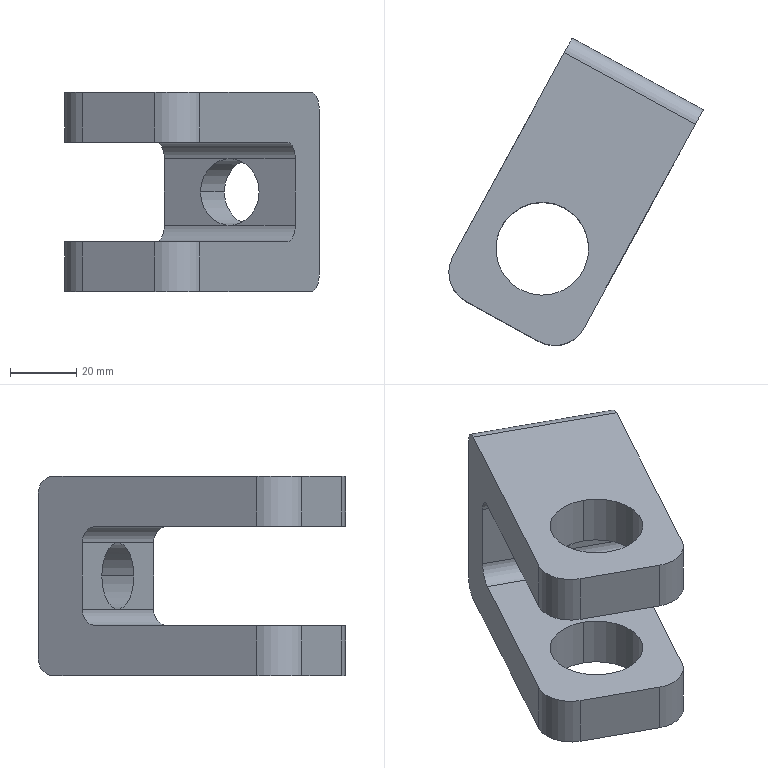Component | SolidWorks | SC-80X130-S-BCylinderY-Joint-1 | 1 solid | 25 faces | box 76.65 x 92.6 x 60 mm | volume 110480 mm3 | cylinder 14 | plane 11 | commonest cylinder face diameters 28 x4 10 x4 20 x4 20.1 x2
STEP:
#1=CARTESIAN_POINT('',(-14.174,0.0304,35.433));
#2=VERTEX_POINT('',#1);
#3=CARTESIAN_POINT('',(-13.862,-0.1403,35.827));
#4=VERTEX_POINT('',#3);
#5=CARTESIAN_POINT('',(-13.827,-0.1591,35.433));
#6=DIRECTION('',(0.479,0.8778,0.));
#7=DIRECTION('',(0.8778,-0.479,0.));
#8=AXIS2_PLACEMENT_3D('',#5,#6,#7);
#9=CIRCLE('',#8,0.3957);
#10=EDGE_CURVE('',#2,#4,#9,.T.);
#11=ORIENTED_EDGE('',*,*,#10,.F.);
#12=CARTESIAN_POINT('',(-13.892,0.5488,35.433));
#13=VERTEX_POINT('',#12);
#14=CARTESIAN_POINT('',(-13.892,0.5488,35.433));
#15=DIRECTION('',(0.479,0.8778,0.));
#16=VECTOR('',#15,39.37);
#17=LINE('',#14,#16);
#18=EDGE_CURVE('',#2,#13,#17,.T.);
#19=ORIENTED_EDGE('',*,*,#18,.T.);
#20=CARTESIAN_POINT('',(-13.197,0.1697,35.433));
#21=VERTEX_POINT('',#20);
#22=CARTESIAN_POINT('',(-13.544,0.3593,35.433));
#23=DIRECTION('',(0.479,0.8778,0.));
#24=DIRECTION('',(0.8778,-0.479,0.));
#25=AXIS2_PLACEMENT_3D('',#22,#23,#24);
#26=CIRCLE('',#25,0.3957);
#27=EDGE_CURVE('',#13,#21,#26,.T.);
#28=ORIENTED_EDGE('',*,*,#27,.T.);
#29=CARTESIAN_POINT('',(-13.48,-0.3487,35.433));
#30=VERTEX_POINT('',#29);
#31=CARTESIAN_POINT('',(-13.197,0.1697,35.433));
#32=DIRECTION('',(0.479,0.8778,0.));
#33=VECTOR('',#32,39.37);
#34=LINE('',#31,#33);
#35=EDGE_CURVE('',#30,#21,#34,.T.);
#36=ORIENTED_EDGE('',*,*,#35,.F.);
#37=CARTESIAN_POINT('',(-13.793,-0.178,35.827));
#38=VERTEX_POINT('',#37);
#39=CARTESIAN_POINT('',(-13.827,-0.1591,35.433));
#40=DIRECTION('',(0.479,0.8778,0.));
#41=DIRECTION('',(0.8778,-0.479,0.));
#42=AXIS2_PLACEMENT_3D('',#39,#40,#41);
#43=CIRCLE('',#42,0.3957);
#44=EDGE_CURVE('',#38,#30,#43,.T.);
#45=ORIENTED_EDGE('',*,*,#44,.F.);
#46=CARTESIAN_POINT('',(-13.862,-0.1403,35.827));
#47=CARTESIAN_POINT('',(-13.839,-0.1528,35.829));
#48=CARTESIAN_POINT('',(-13.816,-0.1654,35.829));
#49=CARTESIAN_POINT('',(-13.793,-0.178,35.827));
#50=B_SPLINE_CURVE_WITH_KNOTS('',3,(#46,#47,#48,#49),.UNSPECIFIED.,.F.,.F.,(4,4),(0.,0.002002),.UNSPECIFIED.);
#51=EDGE_CURVE('',#4,#38,#50,.T.);
#52=ORIENTED_EDGE('',*,*,#51,.F.);
#53=EDGE_LOOP('',(#11,#19,#28,#36,#45,#52));
#54=FACE_OUTER_BOUND('',#53,.T.);
#55=CARTESIAN_POINT('',(-13.544,0.3593,35.433));
#56=DIRECTION('',(0.479,0.8778,0.));
#57=DIRECTION('',(0.8778,-0.479,0.));
#58=AXIS2_PLACEMENT_3D('',#55,#56,#57);
#59=CYLINDRICAL_SURFACE('',#58,0.3957);
#60=ADVANCED_FACE('',(#54),#59,.F.);
#61=CARTESIAN_POINT('',(-14.94,-2.198,34.843));
#62=VERTEX_POINT('',#61);
#63=CARTESIAN_POINT('',(-14.412,-1.23,34.843));
#64=VERTEX_POINT('',#63);
#65=CARTESIAN_POINT('',(-14.676,-1.714,34.843));
#66=DIRECTION('',(-0.,0.,-1.));
#67=DIRECTION('',(0.479,0.8778,0.));
#68=AXIS2_PLACEMENT_3D('',#65,#66,#67);
#69=CIRCLE('',#68,0.5512);
#70=EDGE_CURVE('',#62,#64,#69,.T.);
#71=ORIENTED_EDGE('',*,*,#70,.F.);
#72=CARTESIAN_POINT('',(-14.94,-2.198,34.252));
#73=VERTEX_POINT('',#72);
#74=CARTESIAN_POINT('',(-14.94,-2.198,36.614));
#75=DIRECTION('',(-0.,0.,-1.));
#76=VECTOR('',#75,39.37);
#77=LINE('',#74,#76);
#78=EDGE_CURVE('',#62,#73,#77,.T.);
#79=ORIENTED_EDGE('',*,*,#78,.T.);
#80=CARTESIAN_POINT('',(-14.412,-1.23,34.252));
#81=VERTEX_POINT('',#80);
#82=CARTESIAN_POINT('',(-14.676,-1.714,34.252));
#83=DIRECTION('',(-0.,0.,-1.));
#84=DIRECTION('',(0.479,0.8778,0.));
#85=AXIS2_PLACEMENT_3D('',#82,#83,#84);
#86=CIRCLE('',#85,0.5512);
#87=EDGE_CURVE('',#73,#81,#86,.T.);
#88=ORIENTED_EDGE('',*,*,#87,.T.);
#89=CARTESIAN_POINT('',(-14.412,-1.23,36.614));
#90=DIRECTION('',(-0.,0.,-1.));
#91=VECTOR('',#90,39.37);
#92=LINE('',#89,#91);
#93=EDGE_CURVE('',#64,#81,#92,.T.);
#94=ORIENTED_EDGE('',*,*,#93,.F.);
#95=EDGE_LOOP('',(#71,#79,#88,#94));
#96=FACE_OUTER_BOUND('',#95,.T.);
#97=CARTESIAN_POINT('',(-14.676,-1.714,36.614));
#98=DIRECTION('',(-0.,0.,-1.));
#99=DIRECTION('',(0.479,0.8778,0.));
#100=AXIS2_PLACEMENT_3D('',#97,#98,#99);
#101=CYLINDRICAL_SURFACE('',#100,0.5512);
#102=ADVANCED_FACE('',(#96),#101,.F.);
#103=CARTESIAN_POINT('',(-14.94,-2.198,36.614));
#104=VERTEX_POINT('',#103);
#105=CARTESIAN_POINT('',(-14.412,-1.23,36.614));
#106=VERTEX_POINT('',#105);
#107=CARTESIAN_POINT('',(-14.676,-1.714,36.614));
#108=DIRECTION('',(-0.,0.,-1.));
#109=DIRECTION('',(0.479,0.8778,0.));
#110=AXIS2_PLACEMENT_3D('',#107,#108,#109);
#111=CIRCLE('',#110,0.5512);
#112=EDGE_CURVE('',#104,#106,#111,.T.);
#113=ORIENTED_EDGE('',*,*,#112,.F.);
#114=CARTESIAN_POINT('',(-14.94,-2.198,36.024));
#115=VERTEX_POINT('',#114);
#116=CARTESIAN_POINT('',(-14.94,-2.198,36.614));
#117=DIRECTION('',(-0.,0.,-1.));
#118=VECTOR('',#117,39.37);
#119=LINE('',#116,#118);
#120=EDGE_CURVE('',#104,#115,#119,.T.);
#121=ORIENTED_EDGE('',*,*,#120,.T.);
#122=CARTESIAN_POINT('',(-14.412,-1.23,36.024));
#123=VERTEX_POINT('',#122);
#124=CARTESIAN_POINT('',(-14.676,-1.714,36.024));
#125=DIRECTION('',(0.,-0.,1.));
#126=DIRECTION('',(-0.479,-0.8778,0.));
#127=AXIS2_PLACEMENT_3D('',#124,#125,#126);
#128=CIRCLE('',#127,0.5512);
#129=EDGE_CURVE('',#123,#115,#128,.T.);
#130=ORIENTED_EDGE('',*,*,#129,.F.);
#131=CARTESIAN_POINT('',(-14.412,-1.23,36.614));
#132=DIRECTION('',(-0.,0.,-1.));
#133=VECTOR('',#132,39.37);
#134=LINE('',#131,#133);
#135=EDGE_CURVE('',#106,#123,#134,.T.);
#136=ORIENTED_EDGE('',*,*,#135,.F.);
#137=EDGE_LOOP('',(#113,#121,#130,#136));
#138=FACE_OUTER_BOUND('',#137,.T.);
#139=CARTESIAN_POINT('',(-14.676,-1.714,36.614));
#140=DIRECTION('',(-0.,0.,-1.));
#141=DIRECTION('',(0.479,0.8778,0.));
#142=AXIS2_PLACEMENT_3D('',#139,#140,#141);
#143=CYLINDRICAL_SURFACE('',#142,0.5512);
#144=ADVANCED_FACE('',(#138),#143,.F.);
#145=CARTESIAN_POINT('',(-14.605,0.2652,35.039));
#146=VERTEX_POINT('',#145);
#147=CARTESIAN_POINT('',(-13.862,-0.1403,35.039));
#148=VERTEX_POINT('',#147);
#149=CARTESIAN_POINT('',(-13.05,-0.5835,35.039));
#150=DIRECTION('',(0.8778,-0.479,-0.));
#151=VECTOR('',#150,39.37);
#152=LINE('',#149,#151);
#153=EDGE_CURVE('',#146,#148,#152,.T.);
#154=ORIENTED_EDGE('',*,*,#153,.T.);
#155=CARTESIAN_POINT('',(-13.827,-0.1591,35.433));
#156=DIRECTION('',(0.479,0.8778,0.));
#157=DIRECTION('',(0.8778,-0.479,0.));
#158=AXIS2_PLACEMENT_3D('',#155,#156,#157);
#159=CIRCLE('',#158,0.3957);
#160=EDGE_CURVE('',#148,#2,#159,.T.);
#161=ORIENTED_EDGE('',*,*,#160,.T.);
#162=ORIENTED_EDGE('',*,*,#10,.T.);
#163=CARTESIAN_POINT('',(-14.605,0.2652,35.827));
#164=VERTEX_POINT('',#163);
#165=CARTESIAN_POINT('',(-14.605,0.2652,35.827));
#166=DIRECTION('',(-0.8778,0.479,0.));
#167=VECTOR('',#166,39.37);
#168=LINE('',#165,#167);
#169=EDGE_CURVE('',#4,#164,#168,.T.);
#170=ORIENTED_EDGE('',*,*,#169,.T.);
#171=CARTESIAN_POINT('',(-14.605,0.2652,34.843));
#172=DIRECTION('',(-0.,0.,-1.));
#173=VECTOR('',#172,39.37);
#174=LINE('',#171,#173);
#175=EDGE_CURVE('',#164,#146,#174,.T.);
#176=ORIENTED_EDGE('',*,*,#175,.T.);
#177=EDGE_LOOP('',(#154,#161,#162,#170,#176));
#178=FACE_OUTER_BOUND('',#177,.T.);
#179=CARTESIAN_POINT('',(-13.05,-0.5835,34.843));
#180=DIRECTION('',(0.479,0.8778,0.));
#181=DIRECTION('',(0.8778,-0.479,-0.));
#182=AXIS2_PLACEMENT_3D('',#179,#180,#181);
#183=PLANE('',#182);
#184=ADVANCED_FACE('',(#178),#183,.F.);
#185=CARTESIAN_POINT('',(-14.715,-2.814,36.024));
#186=VERTEX_POINT('',#185);
#187=CARTESIAN_POINT('',(-15.579,-2.343,36.024));
#188=VERTEX_POINT('',#187);
#189=CARTESIAN_POINT('',(-14.37,-3.003,36.024));
#190=DIRECTION('',(-0.8778,0.479,0.));
#191=VECTOR('',#190,39.37);
#192=LINE('',#189,#191);
#193=EDGE_CURVE('',#186,#188,#192,.T.);
#194=ORIENTED_EDGE('',*,*,#193,.F.);
#195=CARTESIAN_POINT('',(-14.715,-2.814,36.614));
#196=VERTEX_POINT('',#195);
#197=CARTESIAN_POINT('',(-14.715,-2.814,36.024));
#198=DIRECTION('',(0.,-0.,1.));
#199=VECTOR('',#198,39.37);
#200=LINE('',#197,#199);
#201=EDGE_CURVE('',#186,#196,#200,.T.);
#202=ORIENTED_EDGE('',*,*,#201,.T.);
#203=CARTESIAN_POINT('',(-15.579,-2.343,36.614));
#204=VERTEX_POINT('',#203);
#205=CARTESIAN_POINT('',(-14.37,-3.003,36.614));
#206=DIRECTION('',(-0.8778,0.479,0.));
#207=VECTOR('',#206,39.37);
#208=LINE('',#205,#207);
#209=EDGE_CURVE('',#196,#204,#208,.T.);
#210=ORIENTED_EDGE('',*,*,#209,.T.);
#211=CARTESIAN_POINT('',(-15.579,-2.343,36.024));
#212=DIRECTION('',(-0.,0.,-1.));
#213=VECTOR('',#212,39.37);
#214=LINE('',#211,#213);
#215=EDGE_CURVE('',#204,#188,#214,.T.);
#216=ORIENTED_EDGE('',*,*,#215,.T.);
#217=EDGE_LOOP('',(#194,#202,#210,#216));
#218=FACE_OUTER_BOUND('',#217,.T.);
#219=CARTESIAN_POINT('',(-14.37,-3.003,36.024));
#220=DIRECTION('',(0.479,0.8778,0.));
#221=DIRECTION('',(0.,-0.,1.));
#222=AXIS2_PLACEMENT_3D('',#219,#220,#221);
#223=PLANE('',#222);
#224=ADVANCED_FACE('',(#218),#223,.F.);
#225=ORIENTED_EDGE('',*,*,#129,.T.);
#226=CARTESIAN_POINT('',(-14.676,-1.714,36.024));
#227=DIRECTION('',(0.,-0.,1.));
#228=DIRECTION('',(-0.479,-0.8778,0.));
#229=AXIS2_PLACEMENT_3D('',#226,#227,#228);
#230=CIRCLE('',#229,0.5512);
#231=EDGE_CURVE('',#115,#123,#230,.T.);
#232=ORIENTED_EDGE('',*,*,#231,.T.);
#233=EDGE_LOOP('',(#225,#232));
#234=FACE_BOUND('',#233,.T.);
#235=CARTESIAN_POINT('',(-14.181,-2.657,36.024));
#236=VERTEX_POINT('',#235);
#237=CARTESIAN_POINT('',(-13.144,-0.7563,36.024));
#238=VERTEX_POINT('',#237);
#239=CARTESIAN_POINT('',(-13.05,-0.5835,36.024));
#240=DIRECTION('',(0.479,0.8778,0.));
#241=VECTOR('',#240,39.37);
#242=LINE('',#239,#241);
#243=EDGE_CURVE('',#236,#238,#242,.T.);
#244=ORIENTED_EDGE('',*,*,#243,.F.);
#245=CARTESIAN_POINT('',(-14.527,-2.468,36.024));
#246=DIRECTION('',(-0.,0.,-1.));
#247=DIRECTION('',(-0.479,-0.8778,0.));
#248=AXIS2_PLACEMENT_3D('',#245,#246,#247);
#249=CIRCLE('',#248,0.3937);
#250=EDGE_CURVE('',#236,#186,#249,.T.);
#251=ORIENTED_EDGE('',*,*,#250,.T.);
#252=ORIENTED_EDGE('',*,*,#193,.T.);
#253=CARTESIAN_POINT('',(-15.736,-1.808,36.024));
#254=VERTEX_POINT('',#253);
#255=CARTESIAN_POINT('',(-15.391,-1.997,36.024));
#256=DIRECTION('',(-0.,0.,-1.));
#257=DIRECTION('',(-0.479,-0.8778,0.));
#258=AXIS2_PLACEMENT_3D('',#255,#256,#257);
#259=CIRCLE('',#258,0.3937);
#260=EDGE_CURVE('',#188,#254,#259,.T.);
#261=ORIENTED_EDGE('',*,*,#260,.T.);
#262=CARTESIAN_POINT('',(-14.699,0.09241,36.024));
#263=VERTEX_POINT('',#262);
#264=CARTESIAN_POINT('',(-14.605,0.2652,36.024));
#265=DIRECTION('',(0.479,0.8778,0.));
#266=VECTOR('',#265,39.37);
#267=LINE('',#264,#266);
#268=EDGE_CURVE('',#254,#263,#267,.T.);
#269=ORIENTED_EDGE('',*,*,#268,.T.);
#270=CARTESIAN_POINT('',(-13.144,-0.7563,36.024));
#271=DIRECTION('',(0.8778,-0.479,-0.));
#272=VECTOR('',#271,39.37);
#273=LINE('',#270,#272);
#274=EDGE_CURVE('',#263,#238,#273,.T.);
#275=ORIENTED_EDGE('',*,*,#274,.T.);
#276=EDGE_LOOP('',(#244,#251,#252,#261,#269,#275));
#277=FACE_OUTER_BOUND('',#276,.T.);
#278=CARTESIAN_POINT('',(-13.05,-0.5835,36.024));
#279=DIRECTION('',(0.,-0.,1.));
#280=DIRECTION('',(-0.479,-0.8778,-0.));
#281=AXIS2_PLACEMENT_3D('',#278,#279,#280);
#282=PLANE('',#281);
#283=ADVANCED_FACE('',(#234,#277),#282,.F.);
#284=CARTESIAN_POINT('',(-13.05,-0.5835,35.827));
#285=VERTEX_POINT('',#284);
#286=CARTESIAN_POINT('',(-14.605,0.2652,35.827));
#287=DIRECTION('',(-0.8778,0.479,0.));
#288=VECTOR('',#287,39.37);
#289=LINE('',#286,#288);
#290=EDGE_CURVE('',#285,#38,#289,.T.);
#291=ORIENTED_EDGE('',*,*,#290,.T.);
#292=ORIENTED_EDGE('',*,*,#44,.T.);
#293=CARTESIAN_POINT('',(-13.793,-0.178,35.039));
#294=VERTEX_POINT('',#293);
#295=CARTESIAN_POINT('',(-13.827,-0.1591,35.433));
#296=DIRECTION('',(0.479,0.8778,0.));
#297=DIRECTION('',(0.8778,-0.479,0.));
#298=AXIS2_PLACEMENT_3D('',#295,#296,#297);
#299=CIRCLE('',#298,0.3957);
#300=EDGE_CURVE('',#30,#294,#299,.T.);
#301=ORIENTED_EDGE('',*,*,#300,.T.);
#302=CARTESIAN_POINT('',(-13.05,-0.5835,35.039));
#303=VERTEX_POINT('',#302);
#304=CARTESIAN_POINT('',(-13.05,-0.5835,35.039));
#305=DIRECTION('',(0.8778,-0.479,-0.));
#306=VECTOR('',#305,39.37);
#307=LINE('',#304,#306);
#308=EDGE_CURVE('',#294,#303,#307,.T.);
#309=ORIENTED_EDGE('',*,*,#308,.T.);
#310=CARTESIAN_POINT('',(-13.05,-0.5835,34.843));
#311=DIRECTION('',(-0.,0.,-1.));
#312=VECTOR('',#311,39.37);
#313=LINE('',#310,#312);
#314=EDGE_CURVE('',#285,#303,#313,.T.);
#315=ORIENTED_EDGE('',*,*,#314,.F.);
#316=EDGE_LOOP('',(#291,#292,#301,#309,#315));
#317=FACE_OUTER_BOUND('',#316,.T.);
#318=CARTESIAN_POINT('',(-13.05,-0.5835,34.843));
#319=DIRECTION('',(0.479,0.8778,0.));
#320=DIRECTION('',(0.8778,-0.479,-0.));
#321=AXIS2_PLACEMENT_3D('',#318,#319,#320);
#322=PLANE('',#321);
#323=ADVANCED_FACE('',(#317),#322,.F.);
#324=CARTESIAN_POINT('',(-14.676,-1.714,34.843));
#325=DIRECTION('',(-0.,0.,-1.));
#326=DIRECTION('',(0.479,0.8778,0.));
#327=AXIS2_PLACEMENT_3D('',#324,#325,#326);
#328=CIRCLE('',#327,0.5512);
#329=EDGE_CURVE('',#64,#62,#328,.T.);
#330=ORIENTED_EDGE('',*,*,#329,.T.);
#331=ORIENTED_EDGE('',*,*,#70,.T.);
#332=EDGE_LOOP('',(#330,#331));
#333=FACE_BOUND('',#332,.T.);
#334=CARTESIAN_POINT('',(-14.715,-2.814,34.843));
#335=VERTEX_POINT('',#334);
#336=CARTESIAN_POINT('',(-15.579,-2.343,34.843));
#337=VERTEX_POINT('',#336);
#338=CARTESIAN_POINT('',(-14.37,-3.003,34.843));
#339=DIRECTION('',(-0.8778,0.479,0.));
#340=VECTOR('',#339,39.37);
#341=LINE('',#338,#340);
#342=EDGE_CURVE('',#335,#337,#341,.T.);
#343=ORIENTED_EDGE('',*,*,#342,.F.);
#344=CARTESIAN_POINT('',(-14.181,-2.657,34.843));
#345=VERTEX_POINT('',#344);
#346=CARTESIAN_POINT('',(-14.527,-2.468,34.843));
#347=DIRECTION('',(0.,-0.,1.));
#348=DIRECTION('',(0.479,0.8778,0.));
#349=AXIS2_PLACEMENT_3D('',#346,#347,#348);
#350=CIRCLE('',#349,0.3937);
#351=EDGE_CURVE('',#335,#345,#350,.T.);
#352=ORIENTED_EDGE('',*,*,#351,.T.);
#353=CARTESIAN_POINT('',(-13.144,-0.7563,34.843));
#354=VERTEX_POINT('',#353);
#355=CARTESIAN_POINT('',(-14.37,-3.003,34.843));
#356=DIRECTION('',(-0.479,-0.8778,-0.));
#357=VECTOR('',#356,39.37);
#358=LINE('',#355,#357);
#359=EDGE_CURVE('',#354,#345,#358,.T.);
#360=ORIENTED_EDGE('',*,*,#359,.F.);
#361=CARTESIAN_POINT('',(-14.699,0.09241,34.843));
#362=VERTEX_POINT('',#361);
#363=CARTESIAN_POINT('',(-14.699,0.09241,34.843));
#364=DIRECTION('',(-0.8778,0.479,0.));
#365=VECTOR('',#364,39.37);
#366=LINE('',#363,#365);
#367=EDGE_CURVE('',#354,#362,#366,.T.);
#368=ORIENTED_EDGE('',*,*,#367,.T.);
#369=CARTESIAN_POINT('',(-15.736,-1.808,34.843));
#370=VERTEX_POINT('',#369);
#371=CARTESIAN_POINT('',(-15.925,-2.154,34.843));
#372=DIRECTION('',(-0.479,-0.8778,-0.));
#373=VECTOR('',#372,39.37);
#374=LINE('',#371,#373);
#375=EDGE_CURVE('',#362,#370,#374,.T.);
#376=ORIENTED_EDGE('',*,*,#375,.T.);
#377=CARTESIAN_POINT('',(-15.391,-1.997,34.843));
#378=DIRECTION('',(0.,-0.,1.));
#379=DIRECTION('',(0.479,0.8778,0.));
#380=AXIS2_PLACEMENT_3D('',#377,#378,#379);
#381=CIRCLE('',#380,0.3937);
#382=EDGE_CURVE('',#370,#337,#381,.T.);
#383=ORIENTED_EDGE('',*,*,#382,.T.);
#384=EDGE_LOOP('',(#343,#352,#360,#368,#376,#383));
#385=FACE_OUTER_BOUND('',#384,.T.);
#386=CARTESIAN_POINT('',(-14.37,-3.003,34.843));
#387=DIRECTION('',(-0.,0.,-1.));
#388=DIRECTION('',(0.479,0.8778,0.));
#389=AXIS2_PLACEMENT_3D('',#386,#387,#388);
#390=PLANE('',#389);
#391=ADVANCED_FACE('',(#333,#385),#390,.F.);
#392=CARTESIAN_POINT('',(-14.715,-2.814,34.252));
#393=VERTEX_POINT('',#392);
#394=CARTESIAN_POINT('',(-15.579,-2.343,34.252));
#395=VERTEX_POINT('',#394);
#396=CARTESIAN_POINT('',(-14.37,-3.003,34.252));
#397=DIRECTION('',(-0.8778,0.479,0.));
#398=VECTOR('',#397,39.37);
#399=LINE('',#396,#398);
#400=EDGE_CURVE('',#393,#395,#399,.T.);
#401=ORIENTED_EDGE('',*,*,#400,.F.);
#402=CARTESIAN_POINT('',(-14.715,-2.814,34.252));
#403=DIRECTION('',(0.,-0.,1.));
#404=VECTOR('',#403,39.37);
#405=LINE('',#402,#404);
#406=EDGE_CURVE('',#393,#335,#405,.T.);
#407=ORIENTED_EDGE('',*,*,#406,.T.);
#408=ORIENTED_EDGE('',*,*,#342,.T.);
#409=CARTESIAN_POINT('',(-15.579,-2.343,34.252));
#410=DIRECTION('',(-0.,0.,-1.));
#411=VECTOR('',#410,39.37);
#412=LINE('',#409,#411);
#413=EDGE_CURVE('',#337,#395,#412,.T.);
#414=ORIENTED_EDGE('',*,*,#413,.T.);
#415=EDGE_LOOP('',(#401,#407,#408,#414));
#416=FACE_OUTER_BOUND('',#415,.T.);
#417=CARTESIAN_POINT('',(-14.37,-3.003,34.252));
#418=DIRECTION('',(0.479,0.8778,0.));
#419=DIRECTION('',(0.,-0.,1.));
#420=AXIS2_PLACEMENT_3D('',#417,#418,#419);
#421=PLANE('',#420);
#422=ADVANCED_FACE('',(#416),#421,.F.);
#423=CARTESIAN_POINT('',(-14.676,-1.714,34.252));
#424=DIRECTION('',(-0.,0.,-1.));
#425=DIRECTION('',(0.479,0.8778,0.));
#426=AXIS2_PLACEMENT_3D('',#423,#424,#425);
#427=CIRCLE('',#426,0.5512);
#428=EDGE_CURVE('',#81,#73,#427,.T.);
#429=ORIENTED_EDGE('',*,*,#428,.F.);
#430=ORIENTED_EDGE('',*,*,#87,.F.);
#431=EDGE_LOOP('',(#429,#430));
#432=FACE_BOUND('',#431,.T.);
#433=CARTESIAN_POINT('',(-14.181,-2.657,34.252));
#434=VERTEX_POINT('',#433);
#435=CARTESIAN_POINT('',(-12.861,-0.2379,34.252));
#436=VERTEX_POINT('',#435);
#437=CARTESIAN_POINT('',(-12.767,-0.06509,34.252));
#438=DIRECTION('',(0.479,0.8778,0.));
#439=VECTOR('',#438,39.37);
#440=LINE('',#437,#439);
#441=EDGE_CURVE('',#434,#436,#440,.T.);
#442=ORIENTED_EDGE('',*,*,#441,.F.);
#443=CARTESIAN_POINT('',(-14.527,-2.468,34.252));
#444=DIRECTION('',(-0.,0.,-1.));
#445=DIRECTION('',(-0.479,-0.8778,0.));
#446=AXIS2_PLACEMENT_3D('',#443,#444,#445);
#447=CIRCLE('',#446,0.3937);
#448=EDGE_CURVE('',#434,#393,#447,.T.);
#449=ORIENTED_EDGE('',*,*,#448,.T.);
#450=ORIENTED_EDGE('',*,*,#400,.T.);
#451=CARTESIAN_POINT('',(-15.736,-1.808,34.252));
#452=VERTEX_POINT('',#451);
#453=CARTESIAN_POINT('',(-15.391,-1.997,34.252));
#454=DIRECTION('',(-0.,0.,-1.));
#455=DIRECTION('',(-0.479,-0.8778,0.));
#456=AXIS2_PLACEMENT_3D('',#453,#454,#455);
#457=CIRCLE('',#456,0.3937);
#458=EDGE_CURVE('',#395,#452,#457,.T.);
#459=ORIENTED_EDGE('',*,*,#458,.T.);
#460=CARTESIAN_POINT('',(-14.416,0.6108,34.252));
#461=VERTEX_POINT('',#460);
#462=CARTESIAN_POINT('',(-14.322,0.7836,34.252));
#463=DIRECTION('',(0.479,0.8778,0.));
#464=VECTOR('',#463,39.37);
#465=LINE('',#462,#464);
#466=EDGE_CURVE('',#452,#461,#465,.T.);
#467=ORIENTED_EDGE('',*,*,#466,.T.);
#468=CARTESIAN_POINT('',(-12.861,-0.2379,34.252));
#469=DIRECTION('',(0.8778,-0.479,-0.));
#470=VECTOR('',#469,39.37);
#471=LINE('',#468,#470);
#472=EDGE_CURVE('',#461,#436,#471,.T.);
#473=ORIENTED_EDGE('',*,*,#472,.T.);
#474=EDGE_LOOP('',(#442,#449,#450,#459,#467,#473));
#475=FACE_OUTER_BOUND('',#474,.T.);
#476=CARTESIAN_POINT('',(-12.767,-0.06509,34.252));
#477=DIRECTION('',(0.,-0.,1.));
#478=DIRECTION('',(-0.479,-0.8778,-0.));
#479=AXIS2_PLACEMENT_3D('',#476,#477,#478);
#480=PLANE('',#479);
#481=ADVANCED_FACE('',(#432,#475),#480,.F.);
#482=CARTESIAN_POINT('',(-13.544,0.3593,35.433));
#483=DIRECTION('',(0.479,0.8778,0.));
#484=DIRECTION('',(0.8778,-0.479,0.));
#485=AXIS2_PLACEMENT_3D('',#482,#483,#484);
#486=CIRCLE('',#485,0.3957);
#487=EDGE_CURVE('',#21,#13,#486,.T.);
#488=ORIENTED_EDGE('',*,*,#487,.F.);
#489=ORIENTED_EDGE('',*,*,#27,.F.);
#490=EDGE_LOOP('',(#488,#489));
#491=FACE_BOUND('',#490,.T.);
#492=CARTESIAN_POINT('',(-14.322,0.7836,34.449));
#493=VERTEX_POINT('',#492);
#494=CARTESIAN_POINT('',(-14.322,0.7836,36.417));
#495=VERTEX_POINT('',#494);
#496=CARTESIAN_POINT('',(-14.322,0.7836,36.614));
#497=DIRECTION('',(0.,-0.,1.));
#498=VECTOR('',#497,39.37);
#499=LINE('',#496,#498);
#500=EDGE_CURVE('',#493,#495,#499,.T.);
#501=ORIENTED_EDGE('',*,*,#500,.T.);
#502=CARTESIAN_POINT('',(-12.767,-0.06509,36.417));
#503=VERTEX_POINT('',#502);
#504=CARTESIAN_POINT('',(-12.767,-0.06509,36.417));
#505=DIRECTION('',(0.8778,-0.479,-0.));
#506=VECTOR('',#505,39.37);
#507=LINE('',#504,#506);
#508=EDGE_CURVE('',#495,#503,#507,.T.);
#509=ORIENTED_EDGE('',*,*,#508,.T.);
#510=CARTESIAN_POINT('',(-12.767,-0.06509,34.449));
#511=VERTEX_POINT('',#510);
#512=CARTESIAN_POINT('',(-12.767,-0.06509,36.614));
#513=DIRECTION('',(0.,-0.,1.));
#514=VECTOR('',#513,39.37);
#515=LINE('',#512,#514);
#516=EDGE_CURVE('',#511,#503,#515,.T.);
#517=ORIENTED_EDGE('',*,*,#516,.F.);
#518=CARTESIAN_POINT('',(-12.767,-0.06509,34.449));
#519=DIRECTION('',(-0.8778,0.479,0.));
#520=VECTOR('',#519,39.37);
#521=LINE('',#518,#520);
#522=EDGE_CURVE('',#511,#493,#521,.T.);
#523=ORIENTED_EDGE('',*,*,#522,.T.);
#524=EDGE_LOOP('',(#501,#509,#517,#523));
#525=FACE_OUTER_BOUND('',#524,.T.);
#526=CARTESIAN_POINT('',(-12.767,-0.06509,36.614));
#527=DIRECTION('',(-0.479,-0.8778,-0.));
#528=DIRECTION('',(-0.8778,0.479,0.));
#529=AXIS2_PLACEMENT_3D('',#526,#527,#528);
#530=PLANE('',#529);
#531=ADVANCED_FACE('',(#491,#525),#530,.F.);
#532=CARTESIAN_POINT('',(-14.676,-1.714,36.614));
#533=DIRECTION('',(-0.,0.,-1.));
#534=DIRECTION('',(0.479,0.8778,0.));
#535=AXIS2_PLACEMENT_3D('',#532,#533,#534);
#536=CIRCLE('',#535,0.5512);
#537=EDGE_CURVE('',#106,#104,#536,.T.);
#538=ORIENTED_EDGE('',*,*,#537,.T.);
#539=ORIENTED_EDGE('',*,*,#112,.T.);
#540=EDGE_LOOP('',(#538,#539));
#541=FACE_BOUND('',#540,.T.);
#542=ORIENTED_EDGE('',*,*,#209,.F.);
#543=CARTESIAN_POINT('',(-14.181,-2.657,36.614));
#544=VERTEX_POINT('',#543);
#545=CARTESIAN_POINT('',(-14.527,-2.468,36.614));
#546=DIRECTION('',(0.,-0.,1.));
#547=DIRECTION('',(-0.8778,0.479,0.));
#548=AXIS2_PLACEMENT_3D('',#545,#546,#547);
#549=CIRCLE('',#548,0.3937);
#550=EDGE_CURVE('',#196,#544,#549,.T.);
#551=ORIENTED_EDGE('',*,*,#550,.T.);
#552=CARTESIAN_POINT('',(-12.861,-0.2379,36.614));
#553=VERTEX_POINT('',#552);
#554=CARTESIAN_POINT('',(-14.37,-3.003,36.614));
#555=DIRECTION('',(-0.479,-0.8778,-0.));
#556=VECTOR('',#555,39.37);
#557=LINE('',#554,#556);
#558=EDGE_CURVE('',#553,#544,#557,.T.);
#559=ORIENTED_EDGE('',*,*,#558,.F.);
#560=CARTESIAN_POINT('',(-14.416,0.6108,36.614));
#561=VERTEX_POINT('',#560);
#562=CARTESIAN_POINT('',(-12.861,-0.2379,36.614));
#563=DIRECTION('',(-0.8778,0.479,0.));
#564=VECTOR('',#563,39.37);
#565=LINE('',#562,#564);
#566=EDGE_CURVE('',#553,#561,#565,.T.);
#567=ORIENTED_EDGE('',*,*,#566,.T.);
#568=CARTESIAN_POINT('',(-15.736,-1.808,36.614));
#569=VERTEX_POINT('',#568);
#570=CARTESIAN_POINT('',(-15.925,-2.154,36.614));
#571=DIRECTION('',(-0.479,-0.8778,-0.));
#572=VECTOR('',#571,39.37);
#573=LINE('',#570,#572);
#574=EDGE_CURVE('',#561,#569,#573,.T.);
#575=ORIENTED_EDGE('',*,*,#574,.T.);
#576=CARTESIAN_POINT('',(-15.391,-1.997,36.614));
#577=DIRECTION('',(0.,-0.,1.));
#578=DIRECTION('',(-0.8778,0.479,0.));
#579=AXIS2_PLACEMENT_3D('',#576,#577,#578);
#580=CIRCLE('',#579,0.3937);
#581=EDGE_CURVE('',#569,#204,#580,.T.);
#582=ORIENTED_EDGE('',*,*,#581,.T.);
#583=EDGE_LOOP('',(#542,#551,#559,#567,#575,#582));
#584=FACE_OUTER_BOUND('',#583,.T.);
#585=CARTESIAN_POINT('',(-14.37,-3.003,36.614));
#586=DIRECTION('',(-0.,0.,-1.));
#587=DIRECTION('',(-0.8778,0.479,0.));
#588=AXIS2_PLACEMENT_3D('',#585,#586,#587);
#589=PLANE('',#588);
#590=ADVANCED_FACE('',(#541,#584),#589,.F.);
#591=ORIENTED_EDGE('',*,*,#558,.T.);
#592=CARTESIAN_POINT('',(-14.181,-2.657,36.614));
#593=DIRECTION('',(-0.,0.,-1.));
#594=VECTOR('',#593,39.37);
#595=LINE('',#592,#594);
#596=EDGE_CURVE('',#544,#236,#595,.T.);
#597=ORIENTED_EDGE('',*,*,#596,.T.);
#598=ORIENTED_EDGE('',*,*,#243,.T.);
#599=CARTESIAN_POINT('',(-13.144,-0.7563,35.827));
#600=DIRECTION('',(-0.8778,0.479,0.));
#601=DIRECTION('',(0.,-0.,1.));
#602=AXIS2_PLACEMENT_3D('',#599,#600,#601);
#603=CIRCLE('',#602,0.1969);
#604=EDGE_CURVE('',#238,#285,#603,.T.);
#605=ORIENTED_EDGE('',*,*,#604,.T.);
#606=ORIENTED_EDGE('',*,*,#314,.T.);
#607=CARTESIAN_POINT('',(-13.144,-0.7563,35.039));
#608=DIRECTION('',(-0.8778,0.479,0.));
#609=DIRECTION('',(0.,-0.,1.));
#610=AXIS2_PLACEMENT_3D('',#607,#608,#609);
#611=CIRCLE('',#610,0.1969);
#612=EDGE_CURVE('',#303,#354,#611,.T.);
#613=ORIENTED_EDGE('',*,*,#612,.T.);
#614=ORIENTED_EDGE('',*,*,#359,.T.);
#615=CARTESIAN_POINT('',(-14.181,-2.657,36.614));
#616=DIRECTION('',(-0.,0.,-1.));
#617=VECTOR('',#616,39.37);
#618=LINE('',#615,#617);
#619=EDGE_CURVE('',#345,#434,#618,.T.);
#620=ORIENTED_EDGE('',*,*,#619,.T.);
#621=ORIENTED_EDGE('',*,*,#441,.T.);
#622=CARTESIAN_POINT('',(-12.861,-0.2379,34.449));
#623=DIRECTION('',(0.8778,-0.479,-0.));
#624=DIRECTION('',(0.,0.,1.));
#625=AXIS2_PLACEMENT_3D('',#622,#623,#624);
#626=CIRCLE('',#625,0.1969);
#627=EDGE_CURVE('',#436,#511,#626,.T.);
#628=ORIENTED_EDGE('',*,*,#627,.T.);
#629=ORIENTED_EDGE('',*,*,#516,.T.);
#630=CARTESIAN_POINT('',(-12.861,-0.2379,36.417));
#631=DIRECTION('',(0.8778,-0.479,-0.));
#632=DIRECTION('',(0.,-0.,1.));
#633=AXIS2_PLACEMENT_3D('',#630,#631,#632);
#634=CIRCLE('',#633,0.1969);
#635=EDGE_CURVE('',#503,#553,#634,.T.);
#636=ORIENTED_EDGE('',*,*,#635,.T.);
#637=EDGE_LOOP('',(#591,#597,#598,#605,#606,#613,#614,#620,#621,#628,#629,#636));
#638=FACE_OUTER_BOUND('',#637,.T.);
#639=CARTESIAN_POINT('',(-14.37,-3.003,36.614));
#640=DIRECTION('',(-0.8778,0.479,0.));
#641=DIRECTION('',(0.,-0.,1.));
#642=AXIS2_PLACEMENT_3D('',#639,#640,#641);
#643=PLANE('',#642);
#644=ADVANCED_FACE('',(#638),#643,.F.);
#645=ORIENTED_EDGE('',*,*,#268,.F.);
#646=CARTESIAN_POINT('',(-15.736,-1.808,36.614));
#647=DIRECTION('',(0.,-0.,1.));
#648=VECTOR('',#647,39.37);
#649=LINE('',#646,#648);
#650=EDGE_CURVE('',#254,#569,#649,.T.);
#651=ORIENTED_EDGE('',*,*,#650,.T.);
#652=ORIENTED_EDGE('',*,*,#574,.F.);
#653=CARTESIAN_POINT('',(-14.416,0.6108,36.417));
#654=DIRECTION('',(-0.8778,0.479,0.));
#655=DIRECTION('',(0.,-0.,1.));
#656=AXIS2_PLACEMENT_3D('',#653,#654,#655);
#657=CIRCLE('',#656,0.1969);
#658=EDGE_CURVE('',#561,#495,#657,.T.);
#659=ORIENTED_EDGE('',*,*,#658,.T.);
#660=ORIENTED_EDGE('',*,*,#500,.F.);
#661=CARTESIAN_POINT('',(-14.416,0.6108,34.449));
#662=DIRECTION('',(-0.8778,0.479,0.));
#663=DIRECTION('',(0.,-0.,1.));
#664=AXIS2_PLACEMENT_3D('',#661,#662,#663);
#665=CIRCLE('',#664,0.1969);
#666=EDGE_CURVE('',#493,#461,#665,.T.);
#667=ORIENTED_EDGE('',*,*,#666,.T.);
#668=ORIENTED_EDGE('',*,*,#466,.F.);
#669=CARTESIAN_POINT('',(-15.736,-1.808,34.843));
#670=DIRECTION('',(0.,-0.,1.));
#671=VECTOR('',#670,39.37);
#672=LINE('',#669,#671);
#673=EDGE_CURVE('',#452,#370,#672,.T.);
#674=ORIENTED_EDGE('',*,*,#673,.T.);
#675=ORIENTED_EDGE('',*,*,#375,.F.);
#676=CARTESIAN_POINT('',(-14.699,0.09241,35.039));
#677=DIRECTION('',(0.8778,-0.479,-0.));
#678=DIRECTION('',(0.,-0.,1.));
#679=AXIS2_PLACEMENT_3D('',#676,#677,#678);
#680=CIRCLE('',#679,0.1969);
#681=EDGE_CURVE('',#362,#146,#680,.T.);
#682=ORIENTED_EDGE('',*,*,#681,.T.);
#683=ORIENTED_EDGE('',*,*,#175,.F.);
#684=CARTESIAN_POINT('',(-14.699,0.09241,35.827));
#685=DIRECTION('',(0.8778,-0.479,-0.));
#686=DIRECTION('',(0.,-0.,1.));
#687=AXIS2_PLACEMENT_3D('',#684,#685,#686);
#688=CIRCLE('',#687,0.1969);
#689=EDGE_CURVE('',#164,#263,#688,.T.);
#690=ORIENTED_EDGE('',*,*,#689,.T.);
#691=EDGE_LOOP('',(#645,#651,#652,#659,#660,#667,#668,#674,#675,#682,#683,#690));
#692=FACE_OUTER_BOUND('',#691,.T.);
#693=CARTESIAN_POINT('',(-15.925,-2.154,36.614));
#694=DIRECTION('',(-0.8778,0.479,0.));
#695=DIRECTION('',(0.,-0.,1.));
#696=AXIS2_PLACEMENT_3D('',#693,#694,#695);
#697=PLANE('',#696);
#698=ADVANCED_FACE('',(#692),#697,.T.);
#699=ORIENTED_EDGE('',*,*,#308,.F.);
#700=CARTESIAN_POINT('',(-13.793,-0.178,35.039));
#701=CARTESIAN_POINT('',(-13.816,-0.1654,35.037));
#702=CARTESIAN_POINT('',(-13.839,-0.1528,35.037));
#703=CARTESIAN_POINT('',(-13.862,-0.1403,35.039));
#704=B_SPLINE_CURVE_WITH_KNOTS('',3,(#700,#701,#702,#703),.UNSPECIFIED.,.F.,.F.,(4,4),(0.,0.002002),.UNSPECIFIED.);
#705=EDGE_CURVE('',#294,#148,#704,.T.);
#706=ORIENTED_EDGE('',*,*,#705,.T.);
#707=ORIENTED_EDGE('',*,*,#153,.F.);
#708=ORIENTED_EDGE('',*,*,#681,.F.);
#709=ORIENTED_EDGE('',*,*,#367,.F.);
#710=ORIENTED_EDGE('',*,*,#612,.F.);
#711=EDGE_LOOP('',(#699,#706,#707,#708,#709,#710));
#712=FACE_OUTER_BOUND('',#711,.T.);
#713=CARTESIAN_POINT('',(-13.144,-0.7563,35.039));
#714=DIRECTION('',(0.8778,-0.479,-0.));
#715=DIRECTION('',(0.,0.,-1.));
#716=AXIS2_PLACEMENT_3D('',#713,#714,#715);
#717=CYLINDRICAL_SURFACE('',#716,0.1969);
#718=ADVANCED_FACE('',(#712),#717,.F.);
#719=ORIENTED_EDGE('',*,*,#169,.F.);
#720=ORIENTED_EDGE('',*,*,#51,.T.);
#721=ORIENTED_EDGE('',*,*,#290,.F.);
#722=ORIENTED_EDGE('',*,*,#604,.F.);
#723=ORIENTED_EDGE('',*,*,#274,.F.);
#724=ORIENTED_EDGE('',*,*,#689,.F.);
#725=EDGE_LOOP('',(#719,#720,#721,#722,#723,#724));
#726=FACE_OUTER_BOUND('',#725,.T.);
#727=CARTESIAN_POINT('',(-13.144,-0.7563,35.827));
#728=DIRECTION('',(0.8778,-0.479,-0.));
#729=DIRECTION('',(0.,0.,-1.));
#730=AXIS2_PLACEMENT_3D('',#727,#728,#729);
#731=CYLINDRICAL_SURFACE('',#730,0.1969);
#732=ADVANCED_FACE('',(#726),#731,.F.);
#733=ORIENTED_EDGE('',*,*,#635,.F.);
#734=ORIENTED_EDGE('',*,*,#508,.F.);
#735=ORIENTED_EDGE('',*,*,#658,.F.);
#736=ORIENTED_EDGE('',*,*,#566,.F.);
#737=EDGE_LOOP('',(#733,#734,#735,#736));
#738=FACE_OUTER_BOUND('',#737,.T.);
#739=CARTESIAN_POINT('',(-12.861,-0.2379,36.417));
#740=DIRECTION('',(-0.8778,0.479,0.));
#741=DIRECTION('',(0.,-0.,1.));
#742=AXIS2_PLACEMENT_3D('',#739,#740,#741);
#743=CYLINDRICAL_SURFACE('',#742,0.1969);
#744=ADVANCED_FACE('',(#738),#743,.T.);
#745=ORIENTED_EDGE('',*,*,#627,.F.);
#746=ORIENTED_EDGE('',*,*,#472,.F.);
#747=ORIENTED_EDGE('',*,*,#666,.F.);
#748=ORIENTED_EDGE('',*,*,#522,.F.);
#749=EDGE_LOOP('',(#745,#746,#747,#748));
#750=FACE_OUTER_BOUND('',#749,.T.);
#751=CARTESIAN_POINT('',(-12.861,-0.2379,34.449));
#752=DIRECTION('',(-0.8778,0.479,0.));
#753=DIRECTION('',(0.,-0.,1.));
#754=AXIS2_PLACEMENT_3D('',#751,#752,#753);
#755=CYLINDRICAL_SURFACE('',#754,0.1969);
#756=ADVANCED_FACE('',(#750),#755,.T.);
#757=ORIENTED_EDGE('',*,*,#120,.F.);
#758=ORIENTED_EDGE('',*,*,#537,.F.);
#759=ORIENTED_EDGE('',*,*,#135,.T.);
#760=ORIENTED_EDGE('',*,*,#231,.F.);
#761=EDGE_LOOP('',(#757,#758,#759,#760));
#762=FACE_OUTER_BOUND('',#761,.T.);
#763=CARTESIAN_POINT('',(-14.676,-1.714,36.614));
#764=DIRECTION('',(-0.,0.,-1.));
#765=DIRECTION('',(0.479,0.8778,0.));
#766=AXIS2_PLACEMENT_3D('',#763,#764,#765);
#767=CYLINDRICAL_SURFACE('',#766,0.5512);
#768=ADVANCED_FACE('',(#762),#767,.F.);
#769=ORIENTED_EDGE('',*,*,#78,.F.);
#770=ORIENTED_EDGE('',*,*,#329,.F.);
#771=ORIENTED_EDGE('',*,*,#93,.T.);
#772=ORIENTED_EDGE('',*,*,#428,.T.);
#773=EDGE_LOOP('',(#769,#770,#771,#772));
#774=FACE_OUTER_BOUND('',#773,.T.);
#775=CARTESIAN_POINT('',(-14.676,-1.714,36.614));
#776=DIRECTION('',(-0.,0.,-1.));
#777=DIRECTION('',(0.479,0.8778,0.));
#778=AXIS2_PLACEMENT_3D('',#775,#776,#777);
#779=CYLINDRICAL_SURFACE('',#778,0.5512);
#780=ADVANCED_FACE('',(#774),#779,.F.);
#781=ORIENTED_EDGE('',*,*,#18,.F.);
#782=ORIENTED_EDGE('',*,*,#160,.F.);
#783=ORIENTED_EDGE('',*,*,#705,.F.);
#784=ORIENTED_EDGE('',*,*,#300,.F.);
#785=ORIENTED_EDGE('',*,*,#35,.T.);
#786=ORIENTED_EDGE('',*,*,#487,.T.);
#787=EDGE_LOOP('',(#781,#782,#783,#784,#785,#786));
#788=FACE_OUTER_BOUND('',#787,.T.);
#789=CARTESIAN_POINT('',(-13.544,0.3593,35.433));
#790=DIRECTION('',(0.479,0.8778,0.));
#791=DIRECTION('',(0.8778,-0.479,0.));
#792=AXIS2_PLACEMENT_3D('',#789,#790,#791);
#793=CYLINDRICAL_SURFACE('',#792,0.3957);
#794=ADVANCED_FACE('',(#788),#793,.F.);
#795=ORIENTED_EDGE('',*,*,#550,.F.);
#796=ORIENTED_EDGE('',*,*,#201,.F.);
#797=ORIENTED_EDGE('',*,*,#250,.F.);
#798=ORIENTED_EDGE('',*,*,#596,.F.);
#799=EDGE_LOOP('',(#795,#796,#797,#798));
#800=FACE_OUTER_BOUND('',#799,.T.);
#801=CARTESIAN_POINT('',(-14.527,-2.468,36.614));
#802=DIRECTION('',(-0.,0.,-1.));
#803=DIRECTION('',(0.479,0.8778,0.));
#804=AXIS2_PLACEMENT_3D('',#801,#802,#803);
#805=CYLINDRICAL_SURFACE('',#804,0.3937);
#806=ADVANCED_FACE('',(#800),#805,.T.);
#807=ORIENTED_EDGE('',*,*,#581,.F.);
#808=ORIENTED_EDGE('',*,*,#650,.F.);
#809=ORIENTED_EDGE('',*,*,#260,.F.);
#810=ORIENTED_EDGE('',*,*,#215,.F.);
#811=EDGE_LOOP('',(#807,#808,#809,#810));
#812=FACE_OUTER_BOUND('',#811,.T.);
#813=CARTESIAN_POINT('',(-15.391,-1.997,36.024));
#814=DIRECTION('',(0.,-0.,1.));
#815=DIRECTION('',(-0.479,-0.8778,0.));
#816=AXIS2_PLACEMENT_3D('',#813,#814,#815);
#817=CYLINDRICAL_SURFACE('',#816,0.3937);
#818=ADVANCED_FACE('',(#812),#817,.T.);
#819=ORIENTED_EDGE('',*,*,#351,.F.);
#820=ORIENTED_EDGE('',*,*,#406,.F.);
#821=ORIENTED_EDGE('',*,*,#448,.F.);
#822=ORIENTED_EDGE('',*,*,#619,.F.);
#823=EDGE_LOOP('',(#819,#820,#821,#822));
#824=FACE_OUTER_BOUND('',#823,.T.);
#825=CARTESIAN_POINT('',(-14.527,-2.468,36.614));
#826=DIRECTION('',(-0.,0.,-1.));
#827=DIRECTION('',(0.479,0.8778,0.));
#828=AXIS2_PLACEMENT_3D('',#825,#826,#827);
#829=CYLINDRICAL_SURFACE('',#828,0.3937);
#830=ADVANCED_FACE('',(#824),#829,.T.);
#831=ORIENTED_EDGE('',*,*,#382,.F.);
#832=ORIENTED_EDGE('',*,*,#673,.F.);
#833=ORIENTED_EDGE('',*,*,#458,.F.);
#834=ORIENTED_EDGE('',*,*,#413,.F.);
#835=EDGE_LOOP('',(#831,#832,#833,#834));
#836=FACE_OUTER_BOUND('',#835,.T.);
#837=CARTESIAN_POINT('',(-15.391,-1.997,34.252));
#838=DIRECTION('',(0.,-0.,1.));
#839=DIRECTION('',(-0.479,-0.8778,0.));
#840=AXIS2_PLACEMENT_3D('',#837,#838,#839);
#841=CYLINDRICAL_SURFACE('',#840,0.3937);
#842=ADVANCED_FACE('',(#836),#841,.T.);
#843=CLOSED_SHELL('',(#60,#102,#144,#184,#224,#283,#323,#391,#422,#481,#531,#590,#644,#698,#718,#732,#744,#756,#768,#780,#794,#806,#818,#830,#842));
#844=MANIFOLD_SOLID_BREP('',#843);
#845=CARTESIAN_POINT('',(0.,0.,0.));
#846=DIRECTION('',(0.,0.,1.));
#847=DIRECTION('',(1.,0.,0.));
#848=AXIS2_PLACEMENT_3D('',#845,#846,#847);
#849=(LENGTH_UNIT()NAMED_UNIT(*)SI_UNIT($,.METRE.));
#850=LENGTH_MEASURE_WITH_UNIT(LENGTH_MEASURE(0.0254),#849);
#851=DIMENSIONAL_EXPONENTS(1.,0.,0.,0.,0.,0.,0.);
#852=(CONVERSION_BASED_UNIT('',#850)LENGTH_UNIT()NAMED_UNIT(#851));
#853=UNCERTAINTY_MEASURE_WITH_UNIT(LENGTH_MEASURE(0.00001),#852,'','');
#854=(NAMED_UNIT(*)PLANE_ANGLE_UNIT()SI_UNIT($,.RADIAN.));
#855=(NAMED_UNIT(*)SI_UNIT($,.STERADIAN.)SOLID_ANGLE_UNIT());
#856=(GEOMETRIC_REPRESENTATION_CONTEXT(3)GLOBAL_UNCERTAINTY_ASSIGNED_CONTEXT((#853))GLOBAL_UNIT_ASSIGNED_CONTEXT((#852,#854,#855))REPRESENTATION_CONTEXT('',''));
#857=ADVANCED_BREP_SHAPE_REPRESENTATION('',(#844,#848),#856);
#858=COLOUR_RGB('',0.7922,0.8196,0.9333);
#859=FILL_AREA_STYLE_COLOUR('',#858);
#860=FILL_AREA_STYLE('',(#859));
#861=SURFACE_STYLE_FILL_AREA(#860);
#862=SURFACE_SIDE_STYLE('',(#861));
#863=SURFACE_STYLE_USAGE(.BOTH.,#862);
#864=PRESENTATION_STYLE_ASSIGNMENT((#863));
#865=STYLED_ITEM('',(#864),#844);
#866=PRESENTATION_LAYER_ASSIGNMENT('','',(#865));
#867=(LENGTH_UNIT()NAMED_UNIT(*)SI_UNIT($,.METRE.));
#868=LENGTH_MEASURE_WITH_UNIT(LENGTH_MEASURE(0.0254),#867);
#869=DIMENSIONAL_EXPONENTS(1.,0.,0.,0.,0.,0.,0.);
#870=(CONVERSION_BASED_UNIT('',#868)LENGTH_UNIT()NAMED_UNIT(#869));
#871=UNCERTAINTY_MEASURE_WITH_UNIT(LENGTH_MEASURE(0.00001),#870,'','');
#872=(NAMED_UNIT(*)PLANE_ANGLE_UNIT()SI_UNIT($,.RADIAN.));
#873=(NAMED_UNIT(*)SI_UNIT($,.STERADIAN.)SOLID_ANGLE_UNIT());
#874=(GEOMETRIC_REPRESENTATION_CONTEXT(3)GLOBAL_UNCERTAINTY_ASSIGNED_CONTEXT((#871))GLOBAL_UNIT_ASSIGNED_CONTEXT((#870,#872,#873))REPRESENTATION_CONTEXT('',''));
#875=MECHANICAL_DESIGN_GEOMETRIC_PRESENTATION_REPRESENTATION('',(#865),#874);